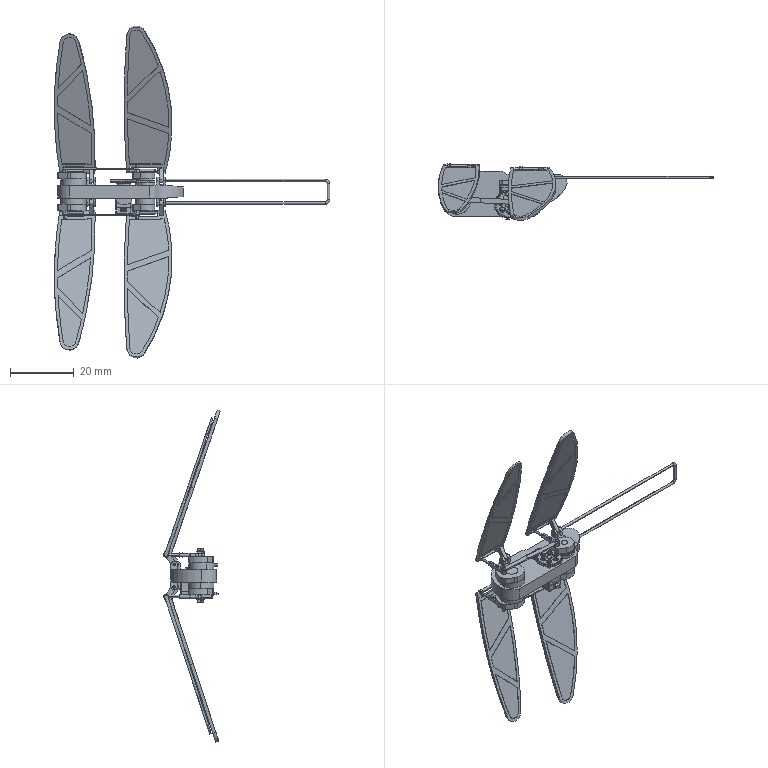Assembly | SolidWorks | mm | 41 component files | 50 solids | 1399 faces | box 86.44 x 17.79 x 104.27 mm | volume 4577 mm3 | cylinder 752 | plane 519 | spline 78 | cone 34 | torus 16 | commonest cylinder face diameters 0.8 x70 1 x70 2.736 x68 1.5 x62 0.1 x52 1.881 x48 0.5 x45 6 x35
Bill of materials:
ConnectingRodRockerArm | 4 |  | Long round rod with a short cylindrical eye boss at one end. The boss has a through hole whose axis is perpendicular to the rod. The rod has a flat along its length and an angled or stepped feature near the far end.
DeflectionCam(Rear) | 2 |  | Thick flat plate shaped like a rounded teardrop or cam, with one straight angled edge. It has one larger through hole and one smaller offset through hole.
EccentricCam(Front) | 2 |  | Flat cam-like or teardrop plate similar to the previous part, but with a much larger central through hole and a small offset through hole.
FrontAxis | 1 |  | Plain solid cylinder with flat end faces.
FrontAxisWasher | 2 |  | Thick flat ring (annular spacer or washer shape) with a central through hole.
FrontWing | 2 |  | Thin, curved, tapering blade-like plate with a rounded tip and a straight root edge. The root edge has small notches and a slot-like recess.
FrontWingYoke | 2 |  | Straight link bar with full-round ends and a through hole at each end.
Fuselage | 1 |  | Elongated plate with an irregular outline. It has a large round hole near one end, a small round hole, a central rectangular through cutout, and two pairs of small tabs with holes that stick out from both faces. It also has a half-round boss on one side and a tapered end.
MG996RServo_stp | 1 | 45 | Rectangular box-shaped housing. One end of the top has a raised round stepped boss with a central bore. A three-conductor lead with a strain-relief-like collar comes out of one end near the bottom, and there are small foot pads at the bottom corners.
Part1^Assembly1 | 2 |  | Long, thin, flat strip link with rounded ends and a small through hole at each end. Part of its length is stepped thinner.
Part25^Assembly1 | 3 |  | Cylindrical pin with chamfered ends and one through cross hole near one end.
Part28^Assembly1 | 1 |  | Flat round washer-like disc with a central through hole. It is thinner, and has a smaller hole relative to its outer diameter, than unnamed part.
Part29^Assembly1 | 1 |  | Thin flat circular disc with a central round through-bore that has one rectangular keyway notch.
Part30^Assembly1 | 1 |  | Short solid prism whose cross-section is a circle with two parallel flats (double-D). It is extruded straight, with plain flat end faces.
Part31^Assembly1 | 1 |  | Short solid prism whose cross-section is a circle with two parallel flats (double-D), with flat end faces. It is similar in form to the other double-flat part.
Part32^Assembly1 | 1 |  | Solid short cylinder with one rectangular axial slot cut into its outer surface along the full length.
Part5^Assembly1 | 1 |  | Solid cylindrical pin with a chamfered edge at one end and a plain square-cut opposite end.
PushRod | 4 |  | Long slender round rod with a split ring at one end, the ring's axis perpendicular to the rod. The opposite end has a small collar or lip.
RearAxis | 1 |  | Long slender solid cylindrical shaft with a short rectangular pocket (keyseat-like recess) near one end.
RearAxisGear | 1 |  | Thin flat spur-gear-like disc with roughly 20-22 teeth around its edge, and a central round bore with one rectangular keyway. It has no hub.
RearAxisWasher | 1 |  | Thick plain ring or spacer: a short cylinder with a concentric round through-bore and flat faces.
RearServoGear | 1 |  | Thin flat spur-gear-like disc with roughly 30 teeth, a small central bore with a keyway notch, and six round lightening holes evenly spaced around the bore.
RearWing | 2 |  | Thin flat plate with an irregular curved, blade- or fin-like outline: one straight edge with a small rectangular notch and a strip-like recess or step, and convex curved edges elsewhere.
RearWingYoke | 2 |  | Flat link bar with a stadium (obround) outline, fully rounded ends, and a round through-hole at each end.
TailWing | 1 |  | Planar U-shaped bent rod (hairpin form): two long, straight, parallel legs of circular cross-section joined at one end by a short straight cross segment, with a rounded bend at each corner. The other ends of the legs are open.
Mates:
1. concentric | Fuselage-1 face at (-10, -2.5, -1) dir (0, 0, 1) r 2 | FrontAxis-2 face at (-10, -2.5, -5) dir (0, 0, 1) r 2
2. width | Fuselage-1 face at (0, 0, 3) dir (0, 0, 1) | Fuselage-1 face at (0, 0, -1) dir (0, 0, -1) | FrontAxis-2 face at (-10, -2.5, -5) dir (0, 0, -1) | FrontAxis-2 face at (-10, -2.5, 7) dir (0, 0, 1)
3. coincident | FrontWing-2 face at (-5.1, 8.619, 8.866) dir (1, 0, 0) | FrontWingYoke-2 face at (-5.1, 6, 4.5) dir (-1, 0, 0)
4. concentric | Fuselage-1 face at (-15, 6, 4.5) dir (1, 0, 0) r 0.4 | FrontWingYoke-2 face at (2.394, 6, 4.5) dir (-1, 0, 0) r 0.4
5. width | Fuselage-1 face at (-3.9, 4.5, 7.5) dir (-1, 0, 0) | Fuselage-1 face at (-5.1, 4.5, 7.5) dir (1, 0, 0) | FrontWingYoke-2 face at (-3.9, 8.092, 6.821) dir (1, 0, 0) | FrontWingYoke-2 face at (-5.1, 6, 4.5) dir (-1, 0, 0)
6. concentric | FrontWing-2 face at (-3.5, 8.396, 7.95) dir (-1, 0, 0) r 0.4 | FrontWingYoke-2 face at (2.394, 8.396, 7.95) dir (-1, 0, 0) r 0.4
7. coincident | EccentricCam(Front)-4 face at (-15.043, -11.49, -5) dir (0, 0, -1) | ConnectingRodRockerArm-4 face at (-12.653, -1.776, -5) dir (0, 0, 1)
8. concentric | ConnectingRodRockerArm-4 face at (-12.653, -0.7263, -5.5) dir (0, 1, 0) r 0.4 | PushRod-4 face at (-12.653, 7.881, -5.5) dir (0, -1, 0) r 0.35
9. width | FrontWing-4 face at (-6.785, 8.226, -4.868) dir (-1, 0, 0) | FrontWing-4 face at (-13.285, 7.599, -6.767) dir (1, 0, 0) | PushRod-4 face at (-12.253, 8.544, -5.5) dir (1, 0, 0) | PushRod-4 face at (-13.053, 8.544, -5.5) dir (-1, 0, 0)
10. coincident | FrontWing-4 face at (-5.1, 7.67, -6.552) dir (1, 0, 0) | FrontWingYoke-4 face at (-5.1, 6, -2.5) dir (-1, 0, 0)
11. concentric | PushRod-4 face at (-13.053, 8.544, -5.5) dir (1, 0, 0) r 0.5 | FrontWing-4 face at (-13.285, 8.544, -5.5) dir (1, 0, 0) r 0.5
12. concentric | FrontWing-4 face at (-3.5, 8.396, -5.95) dir (-1, 0, 0) r 0.4 | FrontWingYoke-4 face at (2.394, 8.396, -5.95) dir (-1, 0, 0) r 0.4
13. width | ConnectingRodRockerArm-4 face at (-12.653, -0.7263, -5.5) dir (0, 1, 0) | ConnectingRodRockerArm-4 face at (-12.653, 4.274, -5.5) dir (0, -1, 0) | PushRod-4 face at (-12.653, 1.031, -5.5) dir (0, -1, 0) | PushRod-4 face at (-12.653, 1.131, -5.5) dir (0, 1, 0)
14. concentric | FrontAxis-2 face at (-10, -2.5, -5) dir (0, 0, 1) r 2 | EccentricCam(Front)-4 face at (-10, -2.5, -5) dir (0, 0, 1) r 2
15. coincident | FrontAxis-2 face at (-10, -2.5, -5) dir (0, 0, -1) | EccentricCam(Front)-4 face at (-15.043, -11.49, -5) dir (0, 0, -1)
16. concentric | Fuselage-1 face at (-15, 6, -2.5) dir (1, 0, 0) r 0.4 | FrontWingYoke-4 face at (2.394, 6, -2.5) dir (-1, 0, 0) r 0.4
17. concentric | FrontAxis-2 face at (-10, -2.5, -5) dir (0, 0, 1) r 2 | FrontAxisWasher-2 face at (-10, -2.5, 5) dir (0, 0, -1) r 2
18. coincident | Fuselage-1 face at (0, 0, 3) dir (0, 0, 1) | FrontAxisWasher-2 face at (-10, -2.5, 3) dir (0, 0, -1)
19. concentric | Fuselage-1 face at (12.5, -3.5, -1) dir (0, 0, 1) r 1 | RearAxis-1 face at (12.5, -3.5, -5) dir (0, 0, 1) r 1
20. width | RearAxis-1 face at (12.5, -3.5, -5) dir (0, 0, -1) | RearAxis-1 face at (12.5, -3.5, 7) dir (0, 0, 1) | Fuselage-1 face at (0, 0, -1) dir (0, 0, -1) | Fuselage-1 face at (0, 0, 3) dir (0, 0, 1)
21. coincident | ConnectingRodRockerArm-2 face at (-12.653, -1.776, 7) dir (0, 0, -1) | EccentricCam(Front)-5 face at (-9.78, 7.805, 7) dir (0, 0, 1)
22. concentric | FrontAxisWasher-2 face at (-10, -2.5, 5) dir (0, 0, -1) r 4 | EccentricCam(Front)-5 face at (-10, -2.5, 7) dir (0, 0, -1) r 2
23. coincident | FrontAxis-2 face at (-10, -2.5, 7) dir (0, 0, 1) | EccentricCam(Front)-5 face at (-9.78, 7.805, 7) dir (0, 0, 1)
24. coincident | EccentricCam(Front)-4 face at (-14.985, 1.522, -5) dir (0.004495, 1, 0) | EccentricCam(Front)-5 face at (-9.809, 1.499, 7) dir (0.004495, 1, 0)
25. concentric | RearAxis-1 face at (12.5, -3.5, -5) dir (0, 0, 1) r 1 | DeflectionCam(Rear)-2 face at (12.5, -3.5, 5) dir (0, 0, 1) r 1
26. coincident | RearAxis-1 face at (12.5, -3.5, 7) dir (0, 0, 1) | DeflectionCam(Rear)-2 face at (12.5, -3.5, 7) dir (0, 0, 1)
27. concentric | DeflectionCam(Rear)-2 face at (9.847, -2.776, 5) dir (0, 0, 1) r 0.5 | Part25^Assembly1-2 face at (9.847, -2.776, 5) dir (0, 0, 1) r 0.5
28. coincident | DeflectionCam(Rear)-2 face at (12.5, -3.5, 5) dir (0, 0, -1) | Part25^Assembly1-2 face at (9.847, -2.776, 5) dir (0, 0, -1)
29. concentric | Part25^Assembly1-2 face at (9.847, -2.776, 5) dir (0, 0, 1) r 0.5 | ConnectingRodRockerArm-10 face at (9.847, -2.776, 7) dir (0, 0, 1) r 0.5
30. coincident | DeflectionCam(Rear)-2 face at (12.5, -3.5, 7) dir (0, 0, 1) | ConnectingRodRockerArm-10 face at (9.847, -2.776, 7) dir (0, 0, -1)
31. concentric | Fuselage-1 face at (15.5, 5, 4.5) dir (1, 0, 0) r 0.4 | RearWingYoke-4 face at (18.1, 5, 4.5) dir (-1, 0, 0) r 0.4
32. coincident | Fuselage-1 face at (18.1, -7.5, 7.7) dir (-1, 0, 0) | RearWingYoke-4 face at (18.1, 5, 4.5) dir (1, 0, 0)
33. concentric | RearWing-2 face at (18.5, 7.398, 7.948) dir (-1, 0, 0) r 0.4 | RearWingYoke-4 face at (18.1, 7.398, 7.948) dir (-1, 0, 0) r 0.4
34. coincident | RearWing-2 face at (16.9, 7.612, 8.867) dir (1, 0, 0) | RearWingYoke-4 face at (16.9, 5, 4.5) dir (-1, 0, 0)
35. concentric | DeflectionCam(Rear)-6 face at (9.847, -2.776, -3) dir (0, 0, -1) r 0.5 | Part25^Assembly1-6 face at (9.847, -2.776, -3) dir (0, 0, -1) r 0.5
36. coincident | DeflectionCam(Rear)-6 face at (12.5, -3.5, -3) dir (0, 0, 1) | Part25^Assembly1-6 face at (9.847, -2.776, -3) dir (0, 0, 1)
37. concentric | ConnectingRodRockerArm-14 face at (9.847, -1.726, -5.5) dir (0, 1, 0) r 0.4 | PushRod-13 face at (9.847, 6.881, -5.5) dir (0, -1, 0) r 0.35
38. concentric | ConnectingRodRockerArm-14 face at (9.847, -2.776, -5) dir (0, 0, -1) r 0.5 | Part25^Assembly1-6 face at (9.847, -2.776, -3) dir (0, 0, -1) r 0.5
39. width | RearWing-5 face at (16.215, 7.226, -4.868) dir (-1, 0, 0) | RearWing-5 face at (7.715, 6.599, -6.767) dir (1, 0, 0) | PushRod-13 face at (10.247, 7.544, -5.5) dir (1, 0, 0) | PushRod-13 face at (9.447, 7.544, -5.5) dir (-1, 0, 0)
40. concentric | PushRod-13 face at (9.447, 7.544, -5.5) dir (1, 0, 0) r 0.5 | RearWing-5 face at (7.715, 7.544, -5.5) dir (1, 0, 0) r 0.5
41. coincident | DeflectionCam(Rear)-6 face at (12.5, -3.5, -5) dir (0, 0, -1) | ConnectingRodRockerArm-14 face at (9.847, -2.776, -5) dir (0, 0, 1)
42. concentric | RearWing-5 face at (18.5, 7.396, -5.95) dir (-1, 0, 0) r 0.4 | RearWingYoke-5 face at (18.1, 7.396, -5.95) dir (-1, 0, 0) r 0.4
43. coincident | RearWing-5 face at (16.9, 6.67, -6.552) dir (1, 0, 0) | RearWingYoke-5 face at (16.9, 5, -2.5) dir (-1, 0, 0)
44. distance | PushRod-13 face at (9.847, 0.031, -5.5) dir (0, -1, 0) | ConnectingRodRockerArm-14 face at (9.847, -1.726, -5.5) dir (0, 1, 0)
45. concentric | RearAxis-1 face at (12.5, -3.5, -5) dir (0, 0, 1) r 1 | DeflectionCam(Rear)-6 face at (12.5, -3.5, -3) dir (0, 0, -1) r 1
46. coincident | RearAxis-1 face at (12.5, -3.5, -5) dir (0, 0, -1) | DeflectionCam(Rear)-6 face at (12.5, -3.5, -5) dir (0, 0, -1)
47. coincident | DeflectionCam(Rear)-2 face at (10.988, -6.091, 5) dir (-0.5039, -0.8638, 0) | DeflectionCam(Rear)-6 face at (10.988, -6.091, -3) dir (-0.5039, -0.8638, 0)
48. concentric | Fuselage-1 face at (9, 5, -2.5) dir (1, 0, 0) r 0.4 | RearWingYoke-5 face at (18.1, 5, -2.5) dir (-1, 0, 0) r 0.4
49. coincident | Fuselage-1 face at (18.1, -7.5, -5.7) dir (-1, 0, 0) | RearWingYoke-5 face at (18.1, 5, -2.5) dir (1, 0, 0)
50. concentric | DeflectionCam(Rear)-2 edge at (12.5, -3.5, 7) dir (0, 0, 1) r 1 | RearAxisGear-2 edge at (12.5, -3.5, 4.5) dir (0, 0, 1) r 1
51. coincident | Fuselage-1 face at (0, 0, 3) dir (0, 0, 1) | MG996RServo_stp-4 face at (3.5, -5.75, 3) dir (0, 0, 1)
52. coincident | Fuselage-1 face at (8.25, 4, -3.5) dir (-1, 0, 0) | MG996RServo_stp-4 face at (8.25, -5.75, 3) dir (1, 0, 0)
53. concentric | RearAxis-1 face at (12.5, -3.5, -5) dir (0, 0, 1) r 1 | RearAxisWasher-2 face at (12.5, -3.5, -1) dir (0, 0, -1) r 1
54. coincident | Fuselage-1 face at (0, 0, -1) dir (0, 0, -1) | RearAxisWasher-2 face at (12.5, -3.5, -1) dir (0, 0, 1)
55. coincident | Fuselage-1 face at (3.25, -6, -3.5) dir (0, 1, 0) | MG996RServo_stp-4 face at (8.25, -6, -4.05) dir (0, -1, 0)
56. coincident | FrontWing-4 face at (-5.1, 7.67, -6.552) dir (1, 0, 0) | FrontWingYoke-4 face at (-5.1, 6, -2.5) dir (-1, 0, 0)
57. gear | RearAxisGear-2 edge at (12.5, -3.5, 4.5) dir (0, 0, 1) r 2.438 | RearServoGear-2 edge at (5.75, -3.5, 4.713) dir (0, 0, 1) r 3.688
58. concentric | RearAxis-1 face at (12.5, -3.5, -5) dir (0, 0, 1) r 1 | Part28^Assembly1-2 face at (12.5, -3.5, 4) dir (0, 0, -1) r 1
59. coincident | Fuselage-1 face at (0, 0, 3) dir (0, 0, 1) | Part28^Assembly1-2 face at (12.5, -3.5, 3) dir (0, 0, -1)
60. concentric | RearAxis-1 face at (12.5, -3.5, -5) dir (0, 0, 1) r 1 | Part29^Assembly1-2 face at (12.5, -3.5, 5) dir (0, 0, -1) r 1
61. coincident | DeflectionCam(Rear)-2 face at (12.5, -3.5, 5) dir (0, 0, -1) | Part29^Assembly1-2 face at (12.5, -3.5, 5) dir (0, 0, 1)
62. coincident | RearAxisGear-2 face at (12.5, -3.5, 4.5) dir (0, 0, 1) | Part29^Assembly1-2 face at (12.5, -3.5, 4.5) dir (0, 0, -1)
63. coincident | RearAxisGear-2 face at (13.678, -4.046, 5) dir (0.1605, 0.987, 0) | Part29^Assembly1-2 face at (13.678, -4.046, 4) dir (0.1605, 0.987, 0)
64. coincident | RearAxis-1 face at (13.79, -3.355, 4) dir (-0.1605, -0.987, 0) | Part29^Assembly1-2 face at (13.79, -3.355, 4) dir (-0.1605, -0.987, 0)
65. coincident | RearAxis-1 face at (13.296, -3.275, 4) dir (0.987, -0.1605, 0) | Part30^Assembly1-4 face at (13.24, -3.62, 4.65) dir (-0.987, 0.1605, 0)
66. coincident | RearAxisGear-2 face at (13.678, -4.046, 5) dir (0.1605, 0.987, 0) | Part30^Assembly1-4 face at (13.678, -4.046, 4.65) dir (-0.1605, -0.987, 0)
67. tangent | RearAxis-1 face at (11.697, -8.435, 5) dir (0, 0, -1) | Part30^Assembly1-4 face at (13.734, -3.701, 4.65) dir (-0.987, 0.1605, 0) r 0.35
68. concentric | ConnectingRodRockerArm-2 face at (-12.653, -1.776, 8) dir (0, 0, -1) r 0.75 | Part1^Assembly1-1 face at (-12.653, -1.776, 8.5) dir (0, 0, -1) r 0.5
69. coincident | ConnectingRodRockerArm-2 face at (-12.653, -1.776, 8) dir (0, 0, 1) | Part1^Assembly1-1 face at (-12.653, -1.776, 8) dir (0, 0, -1)
70. concentric | ConnectingRodRockerArm-4 face at (-12.653, -1.776, -6) dir (0, 0, 1) r 0.75 | Part1^Assembly1-2 face at (-12.653, -1.776, -6) dir (0, 0, -1) r 0.5
71. coincident | ConnectingRodRockerArm-4 face at (-12.653, -1.776, -6) dir (0, 0, -1) | Part1^Assembly1-2 face at (-12.653, -1.776, -6) dir (0, 0, 1)
72. width | FrontWingYoke-4 face at (-3.9, 7.444, -5.271) dir (1, 0, 0) | FrontWingYoke-4 face at (-5.1, 6, -2.5) dir (-1, 0, 0) | Fuselage-1 face at (-3.9, 4.5, -5.5) dir (-1, 0, 0) | Fuselage-1 face at (-5.1, 4.5, -5.5) dir (1, 0, 0)
73. concentric | FrontAxisWasher-3 face at (-10, -2.5, -3) dir (0, 0, 1) r 2 | FrontAxis-2 face at (-10, -2.5, -5) dir (0, 0, 1) r 2
74. coincident | EccentricCam(Front)-4 face at (-15.043, -11.49, -3) dir (0, 0, 1) | FrontAxisWasher-3 face at (-10, -2.5, -3) dir (0, 0, -1)
75. concentric | Part25^Assembly1-2 face at (9.847, -2.776, 9.5) dir (0, 0, 1) r 785.398 | Part1^Assembly1-1 face at (9.847, -2.776, 8.5) dir (0, 0, -1) r 0.5
76. concentric | Part25^Assembly1-6 face at (9.847, -2.776, -3) dir (0, 0, -1) r 0.5 | Part1^Assembly1-2 face at (9.847, -2.776, -6) dir (0, 0, -1) r 0.5
77. coincident | RearServoGear-2 face at (5.63, -4.139, 14.012) dir (0.9782, 0.2075, 0) | Part31^Assembly1-2 face at (5.628, -4.131, 4.562) dir (-0.9782, -0.2075, 0)
78. coincident | MG996RServo_stp-4 face at (5.75, -3.5, 4.013) dir (0, 0, 1) | Part32^Assembly1-2 face at (5.75, -3.5, 4.013) dir (0, 0, -1)
79. concentric | MG996RServo_stp-4 face at (5.75, -3.5, -1.171) dir (0, 0, 1) r 0.75 | Part32^Assembly1-2 face at (5.75, -3.5, 4.812) dir (0, 0, -1) r 0.75
80. coincident | RearServoGear-2 face at (5.75, -3.5, 4.013) dir (0, 0, -1) | MG996RServo_stp-4 face at (5.75, -3.5, 4.013) dir (0, 0, 1)
81. coincident | RearServoGear-2 face at (6.119, -4.035, 14.012) dir (-0.9782, -0.2075, 0) | Part32^Assembly1-2 face at (5.995, -3.448, 4.812) dir (-0.9782, -0.2075, 0)
82. coincident | Part31^Assembly1-2 face at (5.873, -4.08, 4.562) dir (-0.2075, 0.9782, 0) | Part32^Assembly1-2 face at (5.873, -4.08, 4.812) dir (0.2075, -0.9782, 0)
83. tangent | Part31^Assembly1-2 face at (5.873, -4.08, 4.562) dir (0.2075, -0.9782, 0) r 0.25 | Part32^Assembly1-2 face at (5.75, -3.5, 4.812) dir (0, 0, 1)
84. concentric | RearServoGear-2 face at (5.75, -3.5, 4.713) dir (0, 0, -1) r 0.75 | Part32^Assembly1-2 face at (5.75, -3.5, 4.812) dir (0, 0, -1) r 0.75
85. concentric | ConnectingRodRockerArm-2 face at (-12.653, 4.274, 7.5) dir (0, -1, 0) r 0.75 | PushRod-14 face at (-12.653, 7.881, 7.5) dir (0, -1, 0) r 0.35
86. parallel | FrontWing-2 face at (117.269, 2.108, 27.54) dir (0, 0.9459, 0.3245) | RearWing-2 face at (-34.135, 3.151, 21.562) dir (0, 0.9459, 0.3245)
87. concentric | Part1^Assembly1-2 face at (-12.653, -1.776, -6) dir (0, 0, -1) r 0.5 | Part5^Assembly1-4 face at (-12.653, -1.776, -7.5) dir (0, 0, 1) r 0.5
88. coincident | Part25^Assembly1-6 face at (9.847, -2.776, -7.5) dir (0, 0, -1) | Part5^Assembly1-4 face at (-12.653, -1.776, -7.5) dir (0, 0, -1)
89. concentric | Part1^Assembly1-1 face at (-12.653, -1.776, 8.5) dir (0, 0, -1) r 0.5 | Part25^Assembly1-7 face at (-12.653, -1.776, 5) dir (0, 0, 1) r 0.5
90. coincident | Part25^Assembly1-2 face at (9.847, -2.776, 9.5) dir (0, 0, 1) | Part25^Assembly1-7 face at (-12.653, -1.776, 9.5) dir (0, 0, 1)
91. concentric | ConnectingRodRockerArm-10 face at (9.847, 3.274, 7.5) dir (0, -1, 0) r 0.75 | PushRod-15 face at (9.847, 6.889, 7.5) dir (0, -1, 0) r 0.35
92. concentric | RearWing-2 face at (7.715, 7.552, 7.5) dir (1, 0, 0) r 0.5 | PushRod-15 face at (10.247, 7.552, 7.5) dir (-1, 0, 0) r 0.75
93. parallel | FrontWing-4 face at (-14.649, 5.504, -15.975) dir (0, 0.9495, -0.3137) | RearWing-5 face at (-34.135, 3.303, -19.611) dir (0, 0.9495, -0.3137)
94. parallel | FrontWing-2 face at (117.269, 2.108, 27.54) dir (0, 0.9459, 0.3245) | RearWing-2 face at (-34.135, 3.151, 21.562) dir (0, 0.9459, 0.3245)
95. coincident | PushRod-4 face at (-12.653, 1.031, -5.5) dir (0, -1, 0) | PushRod-14 face at (-12.653, 1.031, 7.5) dir (0, -1, 0)
96. concentric | ConnectingRodRockerArm-2 face at (-12.653, -1.776, 8) dir (0, 0, -1) r 0.75 | Part25^Assembly1-7 face at (-12.653, -1.776, 5) dir (0, 0, 1) r 0.5
97. concentric | FrontWing-2 face at (-13.285, 8.544, 7.5) dir (1, 0, 0) r 0.5 | PushRod-14 face at (-12.253, 8.544, 7.5) dir (-1, 0, 0) r 0.75
98. concentric | EccentricCam(Front)-4 face at (-12.653, -1.776, -5) dir (0, 0, 1) r 0.5 | Part5^Assembly1-4 face at (-12.653, -1.776, -7.5) dir (0, 0, 1) r 0.5
99. parallel | FrontWingYoke-4 face at (2.394, 6.657, -2.044) dir (0, 0.8214, 0.5704) | RearWingYoke-5 face at (18.1, 5.616, -2.072) dir (0, 0.8214, 0.5704)